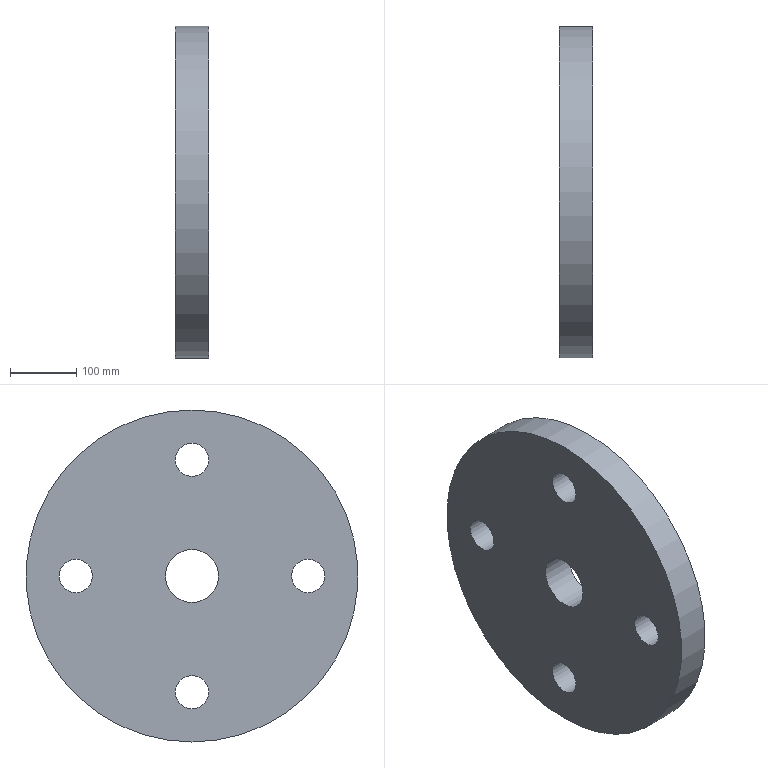Component | NX | OUTER_HAMMER_DISC | 1 solid | 8 faces | box 50 x 500 x 500 mm | volume 9173451 mm3 | cylinder 6 | plane 2 | commonest cylinder face diameters 50 x4 80 x1 500 x1
STEP:
#1=CARTESIAN_POINT('',(0.,0.,0.));
#2=DIRECTION('',(0.,0.,1.));
#3=DIRECTION('',(1.,0.,0.));
#4=AXIS2_PLACEMENT_3D('',#1,#2,#3);
#5=CARTESIAN_POINT('',(719.458,-1343.882,814.997));
#6=VERTEX_POINT('',#5);
#7=CARTESIAN_POINT('',(719.458,-1343.882,839.997));
#8=DIRECTION('',(1.,0.,0.));
#9=DIRECTION('',(0.,0.,-1.));
#10=AXIS2_PLACEMENT_3D('',#7,#8,#9);
#11=CIRCLE('',#10,25.);
#12=CARTESIAN_POINT('',(719.458,-1343.882,839.997));
#13=DIRECTION('',(1.,0.,0.));
#14=DIRECTION('',(0.,0.,-1.));
#15=AXIS2_PLACEMENT_3D('',#12,#13,#14);
#16=CYLINDRICAL_SURFACE('',#15,25.);
#17=CARTESIAN_POINT('',(0.,0.));
#18=DIRECTION('',(1.,0.));
#19=VECTOR('',#18,1.);
#20=LINE('',#17,#19);
#21=(GEOMETRIC_REPRESENTATION_CONTEXT(2)PARAMETRIC_REPRESENTATION_CONTEXT()REPRESENTATION_CONTEXT('',''));
#22=DEFINITIONAL_REPRESENTATION('',(#20),#21);
#23=PCURVE('',#16,#22);
#24=CARTESIAN_POINT('',(719.458,-1081.382,839.997));
#25=DIRECTION('',(1.,0.,0.));
#26=DIRECTION('',(0.,0.,-1.));
#27=AXIS2_PLACEMENT_3D('',#24,#25,#26);
#28=PLANE('',#27);
#29=CARTESIAN_POINT('',(0.,-262.5));
#30=DIRECTION('',(1.,0.));
#31=AXIS2_PLACEMENT_2D('',#29,#30);
#32=CIRCLE('',#31,25.);
#33=(GEOMETRIC_REPRESENTATION_CONTEXT(2)PARAMETRIC_REPRESENTATION_CONTEXT()REPRESENTATION_CONTEXT('',''));
#34=DEFINITIONAL_REPRESENTATION('',(#32),#33);
#35=PCURVE('',#28,#34);
#36=SURFACE_CURVE('',#11,(#23,#35),.PCURVE_S1.);
#37=EDGE_CURVE('',#6,#6,#36,.T.);
#38=ORIENTED_EDGE('',*,*,#37,.T.);
#39=CARTESIAN_POINT('',(769.458,-1343.882,814.997));
#40=VERTEX_POINT('',#39);
#41=CARTESIAN_POINT('',(719.458,-1343.882,814.997));
#42=CARTESIAN_POINT('',(769.458,-1343.882,814.997));
#43=B_SPLINE_CURVE_WITH_KNOTS('',1,(#41,#42),.UNSPECIFIED.,.F.,.F.,(2,2),(0.,50.),.PIECEWISE_BEZIER_KNOTS.);
#44=CARTESIAN_POINT('',(6.283,0.));
#45=DIRECTION('',(0.,1.));
#46=VECTOR('',#45,1.);
#47=LINE('',#44,#46);
#48=(GEOMETRIC_REPRESENTATION_CONTEXT(2)PARAMETRIC_REPRESENTATION_CONTEXT()REPRESENTATION_CONTEXT('',''));
#49=DEFINITIONAL_REPRESENTATION('',(#47),#48);
#50=PCURVE('',#16,#49);
#51=CARTESIAN_POINT('',(0.,0.));
#52=DIRECTION('',(0.,1.));
#53=VECTOR('',#52,1.);
#54=LINE('',#51,#53);
#55=(GEOMETRIC_REPRESENTATION_CONTEXT(2)PARAMETRIC_REPRESENTATION_CONTEXT()REPRESENTATION_CONTEXT('',''));
#56=DEFINITIONAL_REPRESENTATION('',(#54),#55);
#57=PCURVE('',#16,#56);
#58=SEAM_CURVE('',#43,(#50,#57),.PCURVE_S1.);
#59=EDGE_CURVE('',#6,#40,#58,.T.);
#60=ORIENTED_EDGE('',*,*,#59,.T.);
#61=CARTESIAN_POINT('',(769.458,-1343.882,839.997));
#62=DIRECTION('',(1.,0.,0.));
#63=DIRECTION('',(0.,0.,-1.));
#64=AXIS2_PLACEMENT_3D('',#61,#62,#63);
#65=CIRCLE('',#64,25.);
#66=CARTESIAN_POINT('',(0.,50.));
#67=DIRECTION('',(1.,0.));
#68=VECTOR('',#67,1.);
#69=LINE('',#66,#68);
#70=(GEOMETRIC_REPRESENTATION_CONTEXT(2)PARAMETRIC_REPRESENTATION_CONTEXT()REPRESENTATION_CONTEXT('',''));
#71=DEFINITIONAL_REPRESENTATION('',(#69),#70);
#72=PCURVE('',#16,#71);
#73=CARTESIAN_POINT('',(769.458,-1081.382,839.997));
#74=DIRECTION('',(1.,0.,0.));
#75=DIRECTION('',(0.,0.,-1.));
#76=AXIS2_PLACEMENT_3D('',#73,#74,#75);
#77=PLANE('',#76);
#78=CARTESIAN_POINT('',(0.,-262.5));
#79=DIRECTION('',(1.,0.));
#80=AXIS2_PLACEMENT_2D('',#78,#79);
#81=CIRCLE('',#80,25.);
#82=(GEOMETRIC_REPRESENTATION_CONTEXT(2)PARAMETRIC_REPRESENTATION_CONTEXT()REPRESENTATION_CONTEXT('',''));
#83=DEFINITIONAL_REPRESENTATION('',(#81),#82);
#84=PCURVE('',#77,#83);
#85=SURFACE_CURVE('',#65,(#72,#84),.PCURVE_S1.);
#86=EDGE_CURVE('',#40,#40,#85,.T.);
#87=ORIENTED_EDGE('',*,*,#86,.F.);
#88=ORIENTED_EDGE('',*,*,#59,.F.);
#89=EDGE_LOOP('',(#38,#60,#87,#88));
#90=FACE_BOUND('',#89,.F.);
#91=ADVANCED_FACE('',(#90),#16,.F.);
#92=CARTESIAN_POINT('',(719.458,-1143.882,664.997));
#93=VERTEX_POINT('',#92);
#94=CARTESIAN_POINT('',(719.458,-1168.882,664.997));
#95=DIRECTION('',(1.,0.,0.));
#96=DIRECTION('',(0.,1.,0.));
#97=AXIS2_PLACEMENT_3D('',#94,#95,#96);
#98=CIRCLE('',#97,25.);
#99=CARTESIAN_POINT('',(719.458,-1168.882,664.997));
#100=DIRECTION('',(1.,0.,0.));
#101=DIRECTION('',(0.,0.,-1.));
#102=AXIS2_PLACEMENT_3D('',#99,#100,#101);
#103=CYLINDRICAL_SURFACE('',#102,25.);
#104=CARTESIAN_POINT('',(1.571,0.));
#105=DIRECTION('',(1.,0.));
#106=VECTOR('',#105,1.);
#107=LINE('',#104,#106);
#108=(GEOMETRIC_REPRESENTATION_CONTEXT(2)PARAMETRIC_REPRESENTATION_CONTEXT()REPRESENTATION_CONTEXT('',''));
#109=DEFINITIONAL_REPRESENTATION('',(#107),#108);
#110=PCURVE('',#103,#109);
#111=CARTESIAN_POINT('',(175.,-87.5));
#112=DIRECTION('',(0.,1.));
#113=AXIS2_PLACEMENT_2D('',#111,#112);
#114=CIRCLE('',#113,25.);
#115=(GEOMETRIC_REPRESENTATION_CONTEXT(2)PARAMETRIC_REPRESENTATION_CONTEXT()REPRESENTATION_CONTEXT('',''));
#116=DEFINITIONAL_REPRESENTATION('',(#114),#115);
#117=PCURVE('',#28,#116);
#118=SURFACE_CURVE('',#98,(#110,#117),.PCURVE_S1.);
#119=EDGE_CURVE('',#93,#93,#118,.T.);
#120=ORIENTED_EDGE('',*,*,#119,.T.);
#121=CARTESIAN_POINT('',(769.458,-1143.882,664.997));
#122=VERTEX_POINT('',#121);
#123=CARTESIAN_POINT('',(719.458,-1143.882,664.997));
#124=CARTESIAN_POINT('',(769.458,-1143.882,664.997));
#125=B_SPLINE_CURVE_WITH_KNOTS('',1,(#123,#124),.UNSPECIFIED.,.F.,.F.,(2,2),(0.,50.),.PIECEWISE_BEZIER_KNOTS.);
#126=CARTESIAN_POINT('',(7.854,0.));
#127=DIRECTION('',(0.,1.));
#128=VECTOR('',#127,1.);
#129=LINE('',#126,#128);
#130=(GEOMETRIC_REPRESENTATION_CONTEXT(2)PARAMETRIC_REPRESENTATION_CONTEXT()REPRESENTATION_CONTEXT('',''));
#131=DEFINITIONAL_REPRESENTATION('',(#129),#130);
#132=PCURVE('',#103,#131);
#133=CARTESIAN_POINT('',(1.571,0.));
#134=DIRECTION('',(0.,1.));
#135=VECTOR('',#134,1.);
#136=LINE('',#133,#135);
#137=(GEOMETRIC_REPRESENTATION_CONTEXT(2)PARAMETRIC_REPRESENTATION_CONTEXT()REPRESENTATION_CONTEXT('',''));
#138=DEFINITIONAL_REPRESENTATION('',(#136),#137);
#139=PCURVE('',#103,#138);
#140=SEAM_CURVE('',#125,(#132,#139),.PCURVE_S1.);
#141=EDGE_CURVE('',#93,#122,#140,.T.);
#142=ORIENTED_EDGE('',*,*,#141,.T.);
#143=CARTESIAN_POINT('',(769.458,-1168.882,664.997));
#144=DIRECTION('',(1.,0.,0.));
#145=DIRECTION('',(0.,1.,0.));
#146=AXIS2_PLACEMENT_3D('',#143,#144,#145);
#147=CIRCLE('',#146,25.);
#148=CARTESIAN_POINT('',(1.571,50.));
#149=DIRECTION('',(1.,0.));
#150=VECTOR('',#149,1.);
#151=LINE('',#148,#150);
#152=(GEOMETRIC_REPRESENTATION_CONTEXT(2)PARAMETRIC_REPRESENTATION_CONTEXT()REPRESENTATION_CONTEXT('',''));
#153=DEFINITIONAL_REPRESENTATION('',(#151),#152);
#154=PCURVE('',#103,#153);
#155=CARTESIAN_POINT('',(175.,-87.5));
#156=DIRECTION('',(0.,1.));
#157=AXIS2_PLACEMENT_2D('',#155,#156);
#158=CIRCLE('',#157,25.);
#159=(GEOMETRIC_REPRESENTATION_CONTEXT(2)PARAMETRIC_REPRESENTATION_CONTEXT()REPRESENTATION_CONTEXT('',''));
#160=DEFINITIONAL_REPRESENTATION('',(#158),#159);
#161=PCURVE('',#77,#160);
#162=SURFACE_CURVE('',#147,(#154,#161),.PCURVE_S1.);
#163=EDGE_CURVE('',#122,#122,#162,.T.);
#164=ORIENTED_EDGE('',*,*,#163,.F.);
#165=ORIENTED_EDGE('',*,*,#141,.F.);
#166=EDGE_LOOP('',(#120,#142,#164,#165));
#167=FACE_BOUND('',#166,.F.);
#168=ADVANCED_FACE('',(#167),#103,.F.);
#169=CARTESIAN_POINT('',(719.458,-1168.882,879.997));
#170=VERTEX_POINT('',#169);
#171=CARTESIAN_POINT('',(719.458,-1168.882,839.997));
#172=DIRECTION('',(1.,0.,0.));
#173=DIRECTION('',(0.,0.,1.));
#174=AXIS2_PLACEMENT_3D('',#171,#172,#173);
#175=CIRCLE('',#174,40.);
#176=CARTESIAN_POINT('',(719.458,-1168.882,839.997));
#177=DIRECTION('',(1.,0.,0.));
#178=DIRECTION('',(0.,0.,-1.));
#179=AXIS2_PLACEMENT_3D('',#176,#177,#178);
#180=CYLINDRICAL_SURFACE('',#179,40.);
#181=CARTESIAN_POINT('',(3.142,0.));
#182=DIRECTION('',(1.,0.));
#183=VECTOR('',#182,1.);
#184=LINE('',#181,#183);
#185=(GEOMETRIC_REPRESENTATION_CONTEXT(2)PARAMETRIC_REPRESENTATION_CONTEXT()REPRESENTATION_CONTEXT('',''));
#186=DEFINITIONAL_REPRESENTATION('',(#184),#185);
#187=PCURVE('',#180,#186);
#188=CARTESIAN_POINT('',(0.,-87.5));
#189=DIRECTION('',(-1.,0.));
#190=AXIS2_PLACEMENT_2D('',#188,#189);
#191=CIRCLE('',#190,40.);
#192=(GEOMETRIC_REPRESENTATION_CONTEXT(2)PARAMETRIC_REPRESENTATION_CONTEXT()REPRESENTATION_CONTEXT('',''));
#193=DEFINITIONAL_REPRESENTATION('',(#191),#192);
#194=PCURVE('',#28,#193);
#195=SURFACE_CURVE('',#175,(#187,#194),.PCURVE_S1.);
#196=EDGE_CURVE('',#170,#170,#195,.T.);
#197=ORIENTED_EDGE('',*,*,#196,.T.);
#198=CARTESIAN_POINT('',(769.458,-1168.882,879.997));
#199=VERTEX_POINT('',#198);
#200=CARTESIAN_POINT('',(719.458,-1168.882,879.997));
#201=CARTESIAN_POINT('',(769.458,-1168.882,879.997));
#202=B_SPLINE_CURVE_WITH_KNOTS('',1,(#200,#201),.UNSPECIFIED.,.F.,.F.,(2,2),(0.,50.),.PIECEWISE_BEZIER_KNOTS.);
#203=CARTESIAN_POINT('',(9.425,0.));
#204=DIRECTION('',(0.,1.));
#205=VECTOR('',#204,1.);
#206=LINE('',#203,#205);
#207=(GEOMETRIC_REPRESENTATION_CONTEXT(2)PARAMETRIC_REPRESENTATION_CONTEXT()REPRESENTATION_CONTEXT('',''));
#208=DEFINITIONAL_REPRESENTATION('',(#206),#207);
#209=PCURVE('',#180,#208);
#210=CARTESIAN_POINT('',(3.142,0.));
#211=DIRECTION('',(0.,1.));
#212=VECTOR('',#211,1.);
#213=LINE('',#210,#212);
#214=(GEOMETRIC_REPRESENTATION_CONTEXT(2)PARAMETRIC_REPRESENTATION_CONTEXT()REPRESENTATION_CONTEXT('',''));
#215=DEFINITIONAL_REPRESENTATION('',(#213),#214);
#216=PCURVE('',#180,#215);
#217=SEAM_CURVE('',#202,(#209,#216),.PCURVE_S1.);
#218=EDGE_CURVE('',#170,#199,#217,.T.);
#219=ORIENTED_EDGE('',*,*,#218,.T.);
#220=CARTESIAN_POINT('',(769.458,-1168.882,839.997));
#221=DIRECTION('',(1.,0.,0.));
#222=DIRECTION('',(0.,0.,1.));
#223=AXIS2_PLACEMENT_3D('',#220,#221,#222);
#224=CIRCLE('',#223,40.);
#225=CARTESIAN_POINT('',(3.142,50.));
#226=DIRECTION('',(1.,0.));
#227=VECTOR('',#226,1.);
#228=LINE('',#225,#227);
#229=(GEOMETRIC_REPRESENTATION_CONTEXT(2)PARAMETRIC_REPRESENTATION_CONTEXT()REPRESENTATION_CONTEXT('',''));
#230=DEFINITIONAL_REPRESENTATION('',(#228),#229);
#231=PCURVE('',#180,#230);
#232=CARTESIAN_POINT('',(0.,-87.5));
#233=DIRECTION('',(-1.,0.));
#234=AXIS2_PLACEMENT_2D('',#232,#233);
#235=CIRCLE('',#234,40.);
#236=(GEOMETRIC_REPRESENTATION_CONTEXT(2)PARAMETRIC_REPRESENTATION_CONTEXT()REPRESENTATION_CONTEXT('',''));
#237=DEFINITIONAL_REPRESENTATION('',(#235),#236);
#238=PCURVE('',#77,#237);
#239=SURFACE_CURVE('',#224,(#231,#238),.PCURVE_S1.);
#240=EDGE_CURVE('',#199,#199,#239,.T.);
#241=ORIENTED_EDGE('',*,*,#240,.F.);
#242=ORIENTED_EDGE('',*,*,#218,.F.);
#243=EDGE_LOOP('',(#197,#219,#241,#242));
#244=FACE_BOUND('',#243,.F.);
#245=ADVANCED_FACE('',(#244),#180,.F.);
#246=CARTESIAN_POINT('',(719.458,-993.882,864.997));
#247=VERTEX_POINT('',#246);
#248=CARTESIAN_POINT('',(719.458,-993.882,839.997));
#249=DIRECTION('',(1.,0.,0.));
#250=DIRECTION('',(0.,0.,1.));
#251=AXIS2_PLACEMENT_3D('',#248,#249,#250);
#252=CIRCLE('',#251,25.);
#253=CARTESIAN_POINT('',(719.458,-993.882,839.997));
#254=DIRECTION('',(1.,0.,0.));
#255=DIRECTION('',(0.,0.,-1.));
#256=AXIS2_PLACEMENT_3D('',#253,#254,#255);
#257=CYLINDRICAL_SURFACE('',#256,25.);
#258=CARTESIAN_POINT('',(3.142,0.));
#259=DIRECTION('',(1.,0.));
#260=VECTOR('',#259,1.);
#261=LINE('',#258,#260);
#262=(GEOMETRIC_REPRESENTATION_CONTEXT(2)PARAMETRIC_REPRESENTATION_CONTEXT()REPRESENTATION_CONTEXT('',''));
#263=DEFINITIONAL_REPRESENTATION('',(#261),#262);
#264=PCURVE('',#257,#263);
#265=CARTESIAN_POINT('',(0.,87.5));
#266=DIRECTION('',(-1.,0.));
#267=AXIS2_PLACEMENT_2D('',#265,#266);
#268=CIRCLE('',#267,25.);
#269=(GEOMETRIC_REPRESENTATION_CONTEXT(2)PARAMETRIC_REPRESENTATION_CONTEXT()REPRESENTATION_CONTEXT('',''));
#270=DEFINITIONAL_REPRESENTATION('',(#268),#269);
#271=PCURVE('',#28,#270);
#272=SURFACE_CURVE('',#252,(#264,#271),.PCURVE_S1.);
#273=EDGE_CURVE('',#247,#247,#272,.T.);
#274=ORIENTED_EDGE('',*,*,#273,.T.);
#275=CARTESIAN_POINT('',(769.458,-993.882,864.997));
#276=VERTEX_POINT('',#275);
#277=CARTESIAN_POINT('',(719.458,-993.882,864.997));
#278=CARTESIAN_POINT('',(769.458,-993.882,864.997));
#279=B_SPLINE_CURVE_WITH_KNOTS('',1,(#277,#278),.UNSPECIFIED.,.F.,.F.,(2,2),(0.,50.),.PIECEWISE_BEZIER_KNOTS.);
#280=CARTESIAN_POINT('',(9.425,0.));
#281=DIRECTION('',(0.,1.));
#282=VECTOR('',#281,1.);
#283=LINE('',#280,#282);
#284=(GEOMETRIC_REPRESENTATION_CONTEXT(2)PARAMETRIC_REPRESENTATION_CONTEXT()REPRESENTATION_CONTEXT('',''));
#285=DEFINITIONAL_REPRESENTATION('',(#283),#284);
#286=PCURVE('',#257,#285);
#287=CARTESIAN_POINT('',(3.142,0.));
#288=DIRECTION('',(0.,1.));
#289=VECTOR('',#288,1.);
#290=LINE('',#287,#289);
#291=(GEOMETRIC_REPRESENTATION_CONTEXT(2)PARAMETRIC_REPRESENTATION_CONTEXT()REPRESENTATION_CONTEXT('',''));
#292=DEFINITIONAL_REPRESENTATION('',(#290),#291);
#293=PCURVE('',#257,#292);
#294=SEAM_CURVE('',#279,(#286,#293),.PCURVE_S1.);
#295=EDGE_CURVE('',#247,#276,#294,.T.);
#296=ORIENTED_EDGE('',*,*,#295,.T.);
#297=CARTESIAN_POINT('',(769.458,-993.882,839.997));
#298=DIRECTION('',(1.,0.,0.));
#299=DIRECTION('',(0.,0.,1.));
#300=AXIS2_PLACEMENT_3D('',#297,#298,#299);
#301=CIRCLE('',#300,25.);
#302=CARTESIAN_POINT('',(3.142,50.));
#303=DIRECTION('',(1.,0.));
#304=VECTOR('',#303,1.);
#305=LINE('',#302,#304);
#306=(GEOMETRIC_REPRESENTATION_CONTEXT(2)PARAMETRIC_REPRESENTATION_CONTEXT()REPRESENTATION_CONTEXT('',''));
#307=DEFINITIONAL_REPRESENTATION('',(#305),#306);
#308=PCURVE('',#257,#307);
#309=CARTESIAN_POINT('',(0.,87.5));
#310=DIRECTION('',(-1.,0.));
#311=AXIS2_PLACEMENT_2D('',#309,#310);
#312=CIRCLE('',#311,25.);
#313=(GEOMETRIC_REPRESENTATION_CONTEXT(2)PARAMETRIC_REPRESENTATION_CONTEXT()REPRESENTATION_CONTEXT('',''));
#314=DEFINITIONAL_REPRESENTATION('',(#312),#313);
#315=PCURVE('',#77,#314);
#316=SURFACE_CURVE('',#301,(#308,#315),.PCURVE_S1.);
#317=EDGE_CURVE('',#276,#276,#316,.T.);
#318=ORIENTED_EDGE('',*,*,#317,.F.);
#319=ORIENTED_EDGE('',*,*,#295,.F.);
#320=EDGE_LOOP('',(#274,#296,#318,#319));
#321=FACE_BOUND('',#320,.F.);
#322=ADVANCED_FACE('',(#321),#257,.F.);
#323=CARTESIAN_POINT('',(719.458,-1168.882,1089.997));
#324=VERTEX_POINT('',#323);
#325=CARTESIAN_POINT('',(719.458,-1168.882,839.997));
#326=DIRECTION('',(1.,0.,0.));
#327=DIRECTION('',(0.,0.,1.));
#328=AXIS2_PLACEMENT_3D('',#325,#326,#327);
#329=CIRCLE('',#328,250.);
#330=CARTESIAN_POINT('',(719.458,-1168.882,839.997));
#331=DIRECTION('',(1.,0.,0.));
#332=DIRECTION('',(0.,0.,-1.));
#333=AXIS2_PLACEMENT_3D('',#330,#331,#332);
#334=CYLINDRICAL_SURFACE('',#333,250.);
#335=CARTESIAN_POINT('',(3.142,0.));
#336=DIRECTION('',(1.,0.));
#337=VECTOR('',#336,1.);
#338=LINE('',#335,#337);
#339=(GEOMETRIC_REPRESENTATION_CONTEXT(2)PARAMETRIC_REPRESENTATION_CONTEXT()REPRESENTATION_CONTEXT('',''));
#340=DEFINITIONAL_REPRESENTATION('',(#338),#339);
#341=PCURVE('',#334,#340);
#342=CARTESIAN_POINT('',(0.,-87.5));
#343=DIRECTION('',(-1.,0.));
#344=AXIS2_PLACEMENT_2D('',#342,#343);
#345=CIRCLE('',#344,250.);
#346=(GEOMETRIC_REPRESENTATION_CONTEXT(2)PARAMETRIC_REPRESENTATION_CONTEXT()REPRESENTATION_CONTEXT('',''));
#347=DEFINITIONAL_REPRESENTATION('',(#345),#346);
#348=PCURVE('',#28,#347);
#349=SURFACE_CURVE('',#329,(#341,#348),.PCURVE_S1.);
#350=EDGE_CURVE('',#324,#324,#349,.T.);
#351=ORIENTED_EDGE('',*,*,#350,.T.);
#352=CARTESIAN_POINT('',(769.458,-1168.882,1089.997));
#353=VERTEX_POINT('',#352);
#354=CARTESIAN_POINT('',(719.458,-1168.882,1089.997));
#355=CARTESIAN_POINT('',(769.458,-1168.882,1089.997));
#356=B_SPLINE_CURVE_WITH_KNOTS('',1,(#354,#355),.UNSPECIFIED.,.F.,.F.,(2,2),(0.,50.),.PIECEWISE_BEZIER_KNOTS.);
#357=CARTESIAN_POINT('',(9.425,0.));
#358=DIRECTION('',(0.,1.));
#359=VECTOR('',#358,1.);
#360=LINE('',#357,#359);
#361=(GEOMETRIC_REPRESENTATION_CONTEXT(2)PARAMETRIC_REPRESENTATION_CONTEXT()REPRESENTATION_CONTEXT('',''));
#362=DEFINITIONAL_REPRESENTATION('',(#360),#361);
#363=PCURVE('',#334,#362);
#364=CARTESIAN_POINT('',(3.142,0.));
#365=DIRECTION('',(0.,1.));
#366=VECTOR('',#365,1.);
#367=LINE('',#364,#366);
#368=(GEOMETRIC_REPRESENTATION_CONTEXT(2)PARAMETRIC_REPRESENTATION_CONTEXT()REPRESENTATION_CONTEXT('',''));
#369=DEFINITIONAL_REPRESENTATION('',(#367),#368);
#370=PCURVE('',#334,#369);
#371=SEAM_CURVE('',#356,(#363,#370),.PCURVE_S1.);
#372=EDGE_CURVE('',#324,#353,#371,.T.);
#373=ORIENTED_EDGE('',*,*,#372,.T.);
#374=CARTESIAN_POINT('',(769.458,-1168.882,839.997));
#375=DIRECTION('',(1.,0.,0.));
#376=DIRECTION('',(0.,0.,1.));
#377=AXIS2_PLACEMENT_3D('',#374,#375,#376);
#378=CIRCLE('',#377,250.);
#379=CARTESIAN_POINT('',(3.142,50.));
#380=DIRECTION('',(1.,0.));
#381=VECTOR('',#380,1.);
#382=LINE('',#379,#381);
#383=(GEOMETRIC_REPRESENTATION_CONTEXT(2)PARAMETRIC_REPRESENTATION_CONTEXT()REPRESENTATION_CONTEXT('',''));
#384=DEFINITIONAL_REPRESENTATION('',(#382),#383);
#385=PCURVE('',#334,#384);
#386=CARTESIAN_POINT('',(0.,-87.5));
#387=DIRECTION('',(-1.,0.));
#388=AXIS2_PLACEMENT_2D('',#386,#387);
#389=CIRCLE('',#388,250.);
#390=(GEOMETRIC_REPRESENTATION_CONTEXT(2)PARAMETRIC_REPRESENTATION_CONTEXT()REPRESENTATION_CONTEXT('',''));
#391=DEFINITIONAL_REPRESENTATION('',(#389),#390);
#392=PCURVE('',#77,#391);
#393=SURFACE_CURVE('',#378,(#385,#392),.PCURVE_S1.);
#394=EDGE_CURVE('',#353,#353,#393,.T.);
#395=ORIENTED_EDGE('',*,*,#394,.F.);
#396=ORIENTED_EDGE('',*,*,#372,.F.);
#397=EDGE_LOOP('',(#351,#373,#395,#396));
#398=FACE_BOUND('',#397,.T.);
#399=ADVANCED_FACE('',(#398),#334,.T.);
#400=CARTESIAN_POINT('',(719.458,-1193.882,1014.997));
#401=VERTEX_POINT('',#400);
#402=CARTESIAN_POINT('',(719.458,-1168.882,1014.997));
#403=DIRECTION('',(1.,0.,0.));
#404=DIRECTION('',(0.,-1.,0.));
#405=AXIS2_PLACEMENT_3D('',#402,#403,#404);
#406=CIRCLE('',#405,25.);
#407=CARTESIAN_POINT('',(719.458,-1168.882,1014.997));
#408=DIRECTION('',(1.,0.,0.));
#409=DIRECTION('',(0.,0.,-1.));
#410=AXIS2_PLACEMENT_3D('',#407,#408,#409);
#411=CYLINDRICAL_SURFACE('',#410,25.);
#412=CARTESIAN_POINT('',(4.712,0.));
#413=DIRECTION('',(1.,0.));
#414=VECTOR('',#413,1.);
#415=LINE('',#412,#414);
#416=(GEOMETRIC_REPRESENTATION_CONTEXT(2)PARAMETRIC_REPRESENTATION_CONTEXT()REPRESENTATION_CONTEXT('',''));
#417=DEFINITIONAL_REPRESENTATION('',(#415),#416);
#418=PCURVE('',#411,#417);
#419=CARTESIAN_POINT('',(-175.,-87.5));
#420=DIRECTION('',(0.,-1.));
#421=AXIS2_PLACEMENT_2D('',#419,#420);
#422=CIRCLE('',#421,25.);
#423=(GEOMETRIC_REPRESENTATION_CONTEXT(2)PARAMETRIC_REPRESENTATION_CONTEXT()REPRESENTATION_CONTEXT('',''));
#424=DEFINITIONAL_REPRESENTATION('',(#422),#423);
#425=PCURVE('',#28,#424);
#426=SURFACE_CURVE('',#406,(#418,#425),.PCURVE_S1.);
#427=EDGE_CURVE('',#401,#401,#426,.T.);
#428=ORIENTED_EDGE('',*,*,#427,.T.);
#429=CARTESIAN_POINT('',(769.458,-1193.882,1014.997));
#430=VERTEX_POINT('',#429);
#431=CARTESIAN_POINT('',(719.458,-1193.882,1014.997));
#432=CARTESIAN_POINT('',(769.458,-1193.882,1014.997));
#433=B_SPLINE_CURVE_WITH_KNOTS('',1,(#431,#432),.UNSPECIFIED.,.F.,.F.,(2,2),(0.,50.),.PIECEWISE_BEZIER_KNOTS.);
#434=CARTESIAN_POINT('',(10.996,0.));
#435=DIRECTION('',(0.,1.));
#436=VECTOR('',#435,1.);
#437=LINE('',#434,#436);
#438=(GEOMETRIC_REPRESENTATION_CONTEXT(2)PARAMETRIC_REPRESENTATION_CONTEXT()REPRESENTATION_CONTEXT('',''));
#439=DEFINITIONAL_REPRESENTATION('',(#437),#438);
#440=PCURVE('',#411,#439);
#441=CARTESIAN_POINT('',(4.712,0.));
#442=DIRECTION('',(0.,1.));
#443=VECTOR('',#442,1.);
#444=LINE('',#441,#443);
#445=(GEOMETRIC_REPRESENTATION_CONTEXT(2)PARAMETRIC_REPRESENTATION_CONTEXT()REPRESENTATION_CONTEXT('',''));
#446=DEFINITIONAL_REPRESENTATION('',(#444),#445);
#447=PCURVE('',#411,#446);
#448=SEAM_CURVE('',#433,(#440,#447),.PCURVE_S1.);
#449=EDGE_CURVE('',#401,#430,#448,.T.);
#450=ORIENTED_EDGE('',*,*,#449,.T.);
#451=CARTESIAN_POINT('',(769.458,-1168.882,1014.997));
#452=DIRECTION('',(1.,0.,0.));
#453=DIRECTION('',(0.,-1.,0.));
#454=AXIS2_PLACEMENT_3D('',#451,#452,#453);
#455=CIRCLE('',#454,25.);
#456=CARTESIAN_POINT('',(4.712,50.));
#457=DIRECTION('',(1.,0.));
#458=VECTOR('',#457,1.);
#459=LINE('',#456,#458);
#460=(GEOMETRIC_REPRESENTATION_CONTEXT(2)PARAMETRIC_REPRESENTATION_CONTEXT()REPRESENTATION_CONTEXT('',''));
#461=DEFINITIONAL_REPRESENTATION('',(#459),#460);
#462=PCURVE('',#411,#461);
#463=CARTESIAN_POINT('',(-175.,-87.5));
#464=DIRECTION('',(0.,-1.));
#465=AXIS2_PLACEMENT_2D('',#463,#464);
#466=CIRCLE('',#465,25.);
#467=(GEOMETRIC_REPRESENTATION_CONTEXT(2)PARAMETRIC_REPRESENTATION_CONTEXT()REPRESENTATION_CONTEXT('',''));
#468=DEFINITIONAL_REPRESENTATION('',(#466),#467);
#469=PCURVE('',#77,#468);
#470=SURFACE_CURVE('',#455,(#462,#469),.PCURVE_S1.);
#471=EDGE_CURVE('',#430,#430,#470,.T.);
#472=ORIENTED_EDGE('',*,*,#471,.F.);
#473=ORIENTED_EDGE('',*,*,#449,.F.);
#474=EDGE_LOOP('',(#428,#450,#472,#473));
#475=FACE_BOUND('',#474,.F.);
#476=ADVANCED_FACE('',(#475),#411,.F.);
#477=ORIENTED_EDGE('',*,*,#350,.F.);
#478=EDGE_LOOP('',(#477));
#479=FACE_BOUND('',#478,.T.);
#480=ORIENTED_EDGE('',*,*,#273,.T.);
#481=EDGE_LOOP('',(#480));
#482=FACE_BOUND('',#481,.T.);
#483=ORIENTED_EDGE('',*,*,#196,.T.);
#484=EDGE_LOOP('',(#483));
#485=FACE_BOUND('',#484,.T.);
#486=ORIENTED_EDGE('',*,*,#119,.T.);
#487=EDGE_LOOP('',(#486));
#488=FACE_BOUND('',#487,.T.);
#489=ORIENTED_EDGE('',*,*,#37,.T.);
#490=EDGE_LOOP('',(#489));
#491=FACE_BOUND('',#490,.T.);
#492=ORIENTED_EDGE('',*,*,#427,.T.);
#493=EDGE_LOOP('',(#492));
#494=FACE_BOUND('',#493,.T.);
#495=ADVANCED_FACE('',(#479,#482,#485,#488,#491,#494),#28,.F.);
#496=ORIENTED_EDGE('',*,*,#394,.T.);
#497=EDGE_LOOP('',(#496));
#498=FACE_BOUND('',#497,.T.);
#499=ORIENTED_EDGE('',*,*,#317,.F.);
#500=EDGE_LOOP('',(#499));
#501=FACE_BOUND('',#500,.T.);
#502=ORIENTED_EDGE('',*,*,#240,.F.);
#503=EDGE_LOOP('',(#502));
#504=FACE_BOUND('',#503,.T.);
#505=ORIENTED_EDGE('',*,*,#163,.F.);
#506=EDGE_LOOP('',(#505));
#507=FACE_BOUND('',#506,.T.);
#508=ORIENTED_EDGE('',*,*,#86,.F.);
#509=EDGE_LOOP('',(#508));
#510=FACE_BOUND('',#509,.T.);
#511=ORIENTED_EDGE('',*,*,#471,.F.);
#512=EDGE_LOOP('',(#511));
#513=FACE_BOUND('',#512,.T.);
#514=ADVANCED_FACE('',(#498,#501,#504,#507,#510,#513),#77,.T.);
#515=CLOSED_SHELL('',(#91,#168,#245,#322,#399,#476,#495,#514));
#516=MANIFOLD_SOLID_BREP('',#515);
#517=(LENGTH_UNIT()NAMED_UNIT(*)SI_UNIT(.MILLI.,.METRE.));
#518=UNCERTAINTY_MEASURE_WITH_UNIT(LENGTH_MEASURE(0.00001),#517,'','');
#519=(NAMED_UNIT(*)PLANE_ANGLE_UNIT()SI_UNIT($,.RADIAN.));
#520=(NAMED_UNIT(*)SI_UNIT($,.STERADIAN.)SOLID_ANGLE_UNIT());
#521=(GEOMETRIC_REPRESENTATION_CONTEXT(3)GLOBAL_UNCERTAINTY_ASSIGNED_CONTEXT((#518))GLOBAL_UNIT_ASSIGNED_CONTEXT((#517,#519,#520))REPRESENTATION_CONTEXT('',''));
#522=ADVANCED_BREP_SHAPE_REPRESENTATION('',(#4,#516),#521);